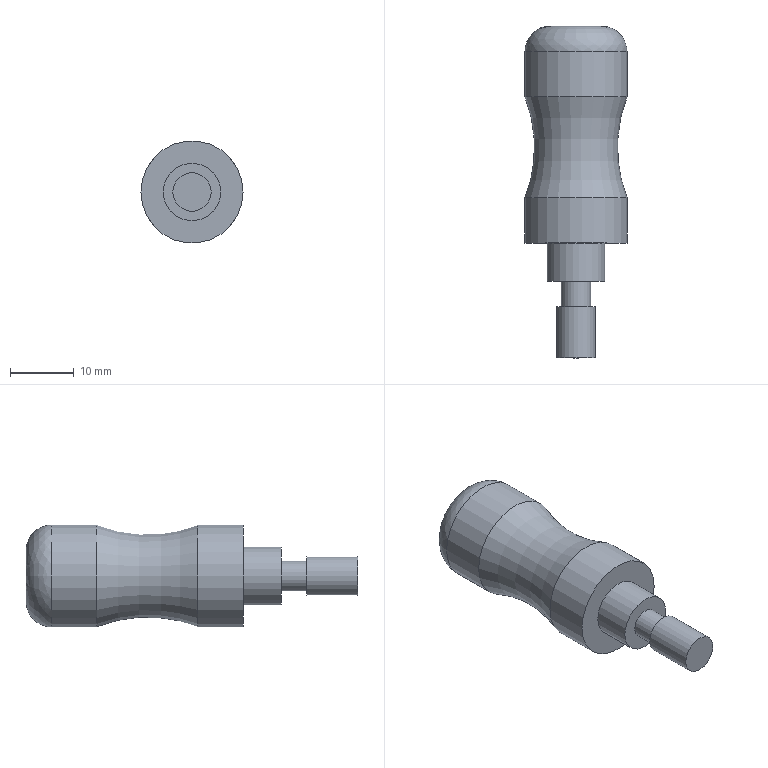Component | NX | 11_HANDLE | 1 solid | 12 faces | box 16 x 52 x 16 mm | volume 6616 mm3 | cylinder 5 | plane 5 | torus 1 | spline 1 | commonest cylinder face diameters 16 x2 9 x1 4.6 x1 6 x1
STEP:
#1=CARTESIAN_POINT('',(0.,0.,0.));
#2=DIRECTION('',(0.,0.,1.));
#3=DIRECTION('',(1.,0.,0.));
#4=AXIS2_PLACEMENT_3D('',#1,#2,#3);
#5=CARTESIAN_POINT('',(10.02,86.13,15.172));
#6=VERTEX_POINT('',#5);
#7=CARTESIAN_POINT('',(2.02,86.13,15.172));
#8=DIRECTION('',(0.,1.,0.));
#9=DIRECTION('',(1.,0.,0.));
#10=AXIS2_PLACEMENT_3D('',#7,#8,#9);
#11=CIRCLE('',#10,8.);
#12=CARTESIAN_POINT('',(2.02,120.13,15.172));
#13=DIRECTION('',(0.,-1.,0.));
#14=DIRECTION('',(1.,0.,0.));
#15=AXIS2_PLACEMENT_3D('',#12,#13,#14);
#16=CYLINDRICAL_SURFACE('',#15,8.);
#17=CARTESIAN_POINT('',(6.283,34.));
#18=DIRECTION('',(-1.,0.));
#19=VECTOR('',#18,1.);
#20=LINE('',#17,#19);
#21=(GEOMETRIC_REPRESENTATION_CONTEXT(2)PARAMETRIC_REPRESENTATION_CONTEXT()REPRESENTATION_CONTEXT('',''));
#22=DEFINITIONAL_REPRESENTATION('',(#20),#21);
#23=PCURVE('',#16,#22);
#24=CARTESIAN_POINT('',(2.02,86.13,15.172));
#25=DIRECTION('',(0.,-1.,0.));
#26=DIRECTION('',(1.,0.,0.));
#27=AXIS2_PLACEMENT_3D('',#24,#25,#26);
#28=PLANE('',#27);
#29=CARTESIAN_POINT('',(8.,0.));
#30=CARTESIAN_POINT('',(8.,-13.856));
#31=CARTESIAN_POINT('',(-4.,-6.928));
#32=CARTESIAN_POINT('',(-16.,-0.));
#33=CARTESIAN_POINT('',(-4.,6.928));
#34=CARTESIAN_POINT('',(8.,13.856));
#35=CARTESIAN_POINT('',(8.,0.));
#36=(BOUNDED_CURVE()B_SPLINE_CURVE(2,(#29,#30,#31,#32,#33,#34,#35),.UNSPECIFIED.,.T.,.F.)B_SPLINE_CURVE_WITH_KNOTS((1,2,2,2,2,1),(-2.094,0.,2.094,4.189,6.283,8.378),.UNSPECIFIED.)CURVE()GEOMETRIC_REPRESENTATION_ITEM()RATIONAL_B_SPLINE_CURVE((1.,0.5,1.,0.5,1.,0.5,1.))REPRESENTATION_ITEM(''));
#37=(GEOMETRIC_REPRESENTATION_CONTEXT(2)PARAMETRIC_REPRESENTATION_CONTEXT()REPRESENTATION_CONTEXT('',''));
#38=DEFINITIONAL_REPRESENTATION('',(#36),#37);
#39=PCURVE('',#28,#38);
#40=SURFACE_CURVE('',#11,(#23,#39),.PCURVE_S1.);
#41=EDGE_CURVE('',#6,#6,#40,.T.);
#42=ORIENTED_EDGE('',*,*,#41,.T.);
#43=CARTESIAN_POINT('',(10.02,93.23,15.172));
#44=VERTEX_POINT('',#43);
#45=CARTESIAN_POINT('',(10.02,93.23,15.172));
#46=CARTESIAN_POINT('',(10.02,86.13,15.172));
#47=B_SPLINE_CURVE_WITH_KNOTS('',1,(#45,#46),.UNSPECIFIED.,.F.,.F.,(2,2),(26.9,34.),.PIECEWISE_BEZIER_KNOTS.);
#48=CARTESIAN_POINT('',(0.,0.));
#49=DIRECTION('',(0.,1.));
#50=VECTOR('',#49,1.);
#51=LINE('',#48,#50);
#52=(GEOMETRIC_REPRESENTATION_CONTEXT(2)PARAMETRIC_REPRESENTATION_CONTEXT()REPRESENTATION_CONTEXT('',''));
#53=DEFINITIONAL_REPRESENTATION('',(#51),#52);
#54=PCURVE('',#16,#53);
#55=CARTESIAN_POINT('',(6.283,0.));
#56=DIRECTION('',(0.,1.));
#57=VECTOR('',#56,1.);
#58=LINE('',#55,#57);
#59=(GEOMETRIC_REPRESENTATION_CONTEXT(2)PARAMETRIC_REPRESENTATION_CONTEXT()REPRESENTATION_CONTEXT('',''));
#60=DEFINITIONAL_REPRESENTATION('',(#58),#59);
#61=PCURVE('',#16,#60);
#62=SEAM_CURVE('',#47,(#54,#61),.PCURVE_S1.);
#63=EDGE_CURVE('',#44,#6,#62,.T.);
#64=ORIENTED_EDGE('',*,*,#63,.F.);
#65=CARTESIAN_POINT('',(-5.98,93.23,15.172));
#66=VERTEX_POINT('',#65);
#67=CARTESIAN_POINT('',(2.02,93.23,15.172));
#68=DIRECTION('',(0.,-1.,0.));
#69=DIRECTION('',(-1.,0.,0.));
#70=AXIS2_PLACEMENT_3D('',#67,#68,#69);
#71=CIRCLE('',#70,8.);
#72=CARTESIAN_POINT('',(-3.142,26.9));
#73=DIRECTION('',(1.,0.));
#74=VECTOR('',#73,1.);
#75=LINE('',#72,#74);
#76=(GEOMETRIC_REPRESENTATION_CONTEXT(2)PARAMETRIC_REPRESENTATION_CONTEXT()REPRESENTATION_CONTEXT('',''));
#77=DEFINITIONAL_REPRESENTATION('',(#75),#76);
#78=PCURVE('',#16,#77);
#79=CARTESIAN_POINT('',(2.02,101.13,15.172));
#80=DIRECTION('',(0.,1.,0.));
#81=DIRECTION('',(-1.,0.,0.));
#82=AXIS2_PLACEMENT_3D('',#79,#80,#81);
#83=TOROIDAL_SURFACE('',#82,28.053,21.553);
#84=CARTESIAN_POINT('',(6.283,3.517));
#85=DIRECTION('',(-1.,0.));
#86=VECTOR('',#85,1.);
#87=LINE('',#84,#86);
#88=(GEOMETRIC_REPRESENTATION_CONTEXT(2)PARAMETRIC_REPRESENTATION_CONTEXT()REPRESENTATION_CONTEXT('',''));
#89=DEFINITIONAL_REPRESENTATION('',(#87),#88);
#90=PCURVE('',#83,#89);
#91=SURFACE_CURVE('',#71,(#78,#90),.PCURVE_S1.);
#92=EDGE_CURVE('',#44,#66,#91,.T.);
#93=ORIENTED_EDGE('',*,*,#92,.T.);
#94=CARTESIAN_POINT('',(2.02,93.23,15.172));
#95=DIRECTION('',(0.,-1.,0.));
#96=DIRECTION('',(-1.,0.,0.));
#97=AXIS2_PLACEMENT_3D('',#94,#95,#96);
#98=CIRCLE('',#97,8.);
#99=CARTESIAN_POINT('',(3.142,26.9));
#100=DIRECTION('',(1.,0.));
#101=VECTOR('',#100,1.);
#102=LINE('',#99,#101);
#103=(GEOMETRIC_REPRESENTATION_CONTEXT(2)PARAMETRIC_REPRESENTATION_CONTEXT()REPRESENTATION_CONTEXT('',''));
#104=DEFINITIONAL_REPRESENTATION('',(#102),#103);
#105=PCURVE('',#16,#104);
#106=CARTESIAN_POINT('',(6.283,3.517));
#107=DIRECTION('',(-1.,0.));
#108=VECTOR('',#107,1.);
#109=LINE('',#106,#108);
#110=(GEOMETRIC_REPRESENTATION_CONTEXT(2)PARAMETRIC_REPRESENTATION_CONTEXT()REPRESENTATION_CONTEXT('',''));
#111=DEFINITIONAL_REPRESENTATION('',(#109),#110);
#112=PCURVE('',#83,#111);
#113=SURFACE_CURVE('',#98,(#105,#112),.PCURVE_S1.);
#114=EDGE_CURVE('',#66,#44,#113,.T.);
#115=ORIENTED_EDGE('',*,*,#114,.T.);
#116=ORIENTED_EDGE('',*,*,#63,.T.);
#117=EDGE_LOOP('',(#42,#64,#93,#115,#116));
#118=FACE_BOUND('',#117,.T.);
#119=ADVANCED_FACE('',(#118),#16,.T.);
#120=CARTESIAN_POINT('',(6.52,86.13,15.172));
#121=VERTEX_POINT('',#120);
#122=CARTESIAN_POINT('',(2.02,86.13,15.172));
#123=DIRECTION('',(0.,-1.,0.));
#124=DIRECTION('',(1.,0.,0.));
#125=AXIS2_PLACEMENT_3D('',#122,#123,#124);
#126=CIRCLE('',#125,4.5);
#127=CARTESIAN_POINT('',(0.,0.));
#128=DIRECTION('',(1.,0.));
#129=AXIS2_PLACEMENT_2D('',#127,#128);
#130=CIRCLE('',#129,4.5);
#131=(GEOMETRIC_REPRESENTATION_CONTEXT(2)PARAMETRIC_REPRESENTATION_CONTEXT()REPRESENTATION_CONTEXT('',''));
#132=DEFINITIONAL_REPRESENTATION('',(#130),#131);
#133=PCURVE('',#28,#132);
#134=CARTESIAN_POINT('',(2.02,86.13,15.172));
#135=DIRECTION('',(0.,-1.,0.));
#136=DIRECTION('',(1.,0.,0.));
#137=AXIS2_PLACEMENT_3D('',#134,#135,#136);
#138=CYLINDRICAL_SURFACE('',#137,4.5);
#139=CARTESIAN_POINT('',(0.,0.));
#140=DIRECTION('',(1.,0.));
#141=VECTOR('',#140,1.);
#142=LINE('',#139,#141);
#143=(GEOMETRIC_REPRESENTATION_CONTEXT(2)PARAMETRIC_REPRESENTATION_CONTEXT()REPRESENTATION_CONTEXT('',''));
#144=DEFINITIONAL_REPRESENTATION('',(#142),#143);
#145=PCURVE('',#138,#144);
#146=SURFACE_CURVE('',#126,(#133,#145),.PCURVE_S1.);
#147=EDGE_CURVE('',#121,#121,#146,.T.);
#148=ORIENTED_EDGE('',*,*,#147,.F.);
#149=EDGE_LOOP('',(#148));
#150=FACE_BOUND('',#149,.T.);
#151=ORIENTED_EDGE('',*,*,#41,.F.);
#152=EDGE_LOOP('',(#151));
#153=FACE_BOUND('',#152,.T.);
#154=ADVANCED_FACE('',(#150,#153),#28,.T.);
#155=CARTESIAN_POINT('',(4.32,80.13,15.172));
#156=VERTEX_POINT('',#155);
#157=CARTESIAN_POINT('',(2.02,80.13,15.172));
#158=DIRECTION('',(0.,-1.,0.));
#159=DIRECTION('',(1.,0.,0.));
#160=AXIS2_PLACEMENT_3D('',#157,#158,#159);
#161=CIRCLE('',#160,2.3);
#162=CARTESIAN_POINT('',(2.02,80.13,15.172));
#163=DIRECTION('',(0.,-1.,0.));
#164=DIRECTION('',(1.,0.,0.));
#165=AXIS2_PLACEMENT_3D('',#162,#163,#164);
#166=PLANE('',#165);
#167=CARTESIAN_POINT('',(0.,0.));
#168=DIRECTION('',(1.,0.));
#169=AXIS2_PLACEMENT_2D('',#167,#168);
#170=CIRCLE('',#169,2.3);
#171=(GEOMETRIC_REPRESENTATION_CONTEXT(2)PARAMETRIC_REPRESENTATION_CONTEXT()REPRESENTATION_CONTEXT('',''));
#172=DEFINITIONAL_REPRESENTATION('',(#170),#171);
#173=PCURVE('',#166,#172);
#174=CARTESIAN_POINT('',(2.02,80.13,15.172));
#175=DIRECTION('',(0.,-1.,0.));
#176=DIRECTION('',(1.,0.,0.));
#177=AXIS2_PLACEMENT_3D('',#174,#175,#176);
#178=CYLINDRICAL_SURFACE('',#177,2.3);
#179=CARTESIAN_POINT('',(0.,0.));
#180=DIRECTION('',(1.,0.));
#181=VECTOR('',#180,1.);
#182=LINE('',#179,#181);
#183=(GEOMETRIC_REPRESENTATION_CONTEXT(2)PARAMETRIC_REPRESENTATION_CONTEXT()REPRESENTATION_CONTEXT('',''));
#184=DEFINITIONAL_REPRESENTATION('',(#182),#183);
#185=PCURVE('',#178,#184);
#186=SURFACE_CURVE('',#161,(#173,#185),.PCURVE_S1.);
#187=EDGE_CURVE('',#156,#156,#186,.T.);
#188=ORIENTED_EDGE('',*,*,#187,.F.);
#189=EDGE_LOOP('',(#188));
#190=FACE_BOUND('',#189,.T.);
#191=CARTESIAN_POINT('',(6.52,80.13,15.172));
#192=VERTEX_POINT('',#191);
#193=CARTESIAN_POINT('',(2.02,80.13,15.172));
#194=DIRECTION('',(0.,1.,0.));
#195=DIRECTION('',(1.,0.,0.));
#196=AXIS2_PLACEMENT_3D('',#193,#194,#195);
#197=CIRCLE('',#196,4.5);
#198=CARTESIAN_POINT('',(4.5,0.));
#199=CARTESIAN_POINT('',(4.5,-7.794));
#200=CARTESIAN_POINT('',(-2.25,-3.897));
#201=CARTESIAN_POINT('',(-9.,-0.));
#202=CARTESIAN_POINT('',(-2.25,3.897));
#203=CARTESIAN_POINT('',(4.5,7.794));
#204=CARTESIAN_POINT('',(4.5,0.));
#205=(BOUNDED_CURVE()B_SPLINE_CURVE(2,(#198,#199,#200,#201,#202,#203,#204),.UNSPECIFIED.,.T.,.F.)B_SPLINE_CURVE_WITH_KNOTS((1,2,2,2,2,1),(-2.094,0.,2.094,4.189,6.283,8.378),.UNSPECIFIED.)CURVE()GEOMETRIC_REPRESENTATION_ITEM()RATIONAL_B_SPLINE_CURVE((1.,0.5,1.,0.5,1.,0.5,1.))REPRESENTATION_ITEM(''));
#206=(GEOMETRIC_REPRESENTATION_CONTEXT(2)PARAMETRIC_REPRESENTATION_CONTEXT()REPRESENTATION_CONTEXT('',''));
#207=DEFINITIONAL_REPRESENTATION('',(#205),#206);
#208=PCURVE('',#166,#207);
#209=CARTESIAN_POINT('',(6.283,6.));
#210=DIRECTION('',(-1.,0.));
#211=VECTOR('',#210,1.);
#212=LINE('',#209,#211);
#213=(GEOMETRIC_REPRESENTATION_CONTEXT(2)PARAMETRIC_REPRESENTATION_CONTEXT()REPRESENTATION_CONTEXT('',''));
#214=DEFINITIONAL_REPRESENTATION('',(#212),#213);
#215=PCURVE('',#138,#214);
#216=SURFACE_CURVE('',#197,(#208,#215),.PCURVE_S1.);
#217=EDGE_CURVE('',#192,#192,#216,.T.);
#218=ORIENTED_EDGE('',*,*,#217,.F.);
#219=EDGE_LOOP('',(#218));
#220=FACE_BOUND('',#219,.T.);
#221=ADVANCED_FACE('',(#190,#220),#166,.T.);
#222=ORIENTED_EDGE('',*,*,#217,.T.);
#223=CARTESIAN_POINT('',(6.52,86.13,15.172));
#224=CARTESIAN_POINT('',(6.52,80.13,15.172));
#225=B_SPLINE_CURVE_WITH_KNOTS('',1,(#223,#224),.UNSPECIFIED.,.F.,.F.,(2,2),(0.,6.),.PIECEWISE_BEZIER_KNOTS.);
#226=CARTESIAN_POINT('',(0.,0.));
#227=DIRECTION('',(0.,1.));
#228=VECTOR('',#227,1.);
#229=LINE('',#226,#228);
#230=(GEOMETRIC_REPRESENTATION_CONTEXT(2)PARAMETRIC_REPRESENTATION_CONTEXT()REPRESENTATION_CONTEXT('',''));
#231=DEFINITIONAL_REPRESENTATION('',(#229),#230);
#232=PCURVE('',#138,#231);
#233=CARTESIAN_POINT('',(6.283,0.));
#234=DIRECTION('',(0.,1.));
#235=VECTOR('',#234,1.);
#236=LINE('',#233,#235);
#237=(GEOMETRIC_REPRESENTATION_CONTEXT(2)PARAMETRIC_REPRESENTATION_CONTEXT()REPRESENTATION_CONTEXT('',''));
#238=DEFINITIONAL_REPRESENTATION('',(#236),#237);
#239=PCURVE('',#138,#238);
#240=SEAM_CURVE('',#225,(#232,#239),.PCURVE_S1.);
#241=EDGE_CURVE('',#121,#192,#240,.T.);
#242=ORIENTED_EDGE('',*,*,#241,.F.);
#243=ORIENTED_EDGE('',*,*,#147,.T.);
#244=ORIENTED_EDGE('',*,*,#241,.T.);
#245=EDGE_LOOP('',(#222,#242,#243,#244));
#246=FACE_BOUND('',#245,.T.);
#247=ADVANCED_FACE('',(#246),#138,.T.);
#248=CARTESIAN_POINT('',(4.32,76.13,15.172));
#249=VERTEX_POINT('',#248);
#250=CARTESIAN_POINT('',(-0.2796,76.13,15.172));
#251=VERTEX_POINT('',#250);
#252=CARTESIAN_POINT('',(2.02,76.13,15.172));
#253=DIRECTION('',(0.,-1.,0.));
#254=DIRECTION('',(-1.,0.,0.));
#255=AXIS2_PLACEMENT_3D('',#252,#253,#254);
#256=CIRCLE('',#255,2.3);
#257=CARTESIAN_POINT('',(-3.142,4.));
#258=DIRECTION('',(1.,0.));
#259=VECTOR('',#258,1.);
#260=LINE('',#257,#259);
#261=(GEOMETRIC_REPRESENTATION_CONTEXT(2)PARAMETRIC_REPRESENTATION_CONTEXT()REPRESENTATION_CONTEXT('',''));
#262=DEFINITIONAL_REPRESENTATION('',(#260),#261);
#263=PCURVE('',#178,#262);
#264=CARTESIAN_POINT('',(2.02,76.13,15.172));
#265=DIRECTION('',(0.,1.,0.));
#266=DIRECTION('',(-1.,0.,0.));
#267=AXIS2_PLACEMENT_3D('',#264,#265,#266);
#268=PLANE('',#267);
#269=CARTESIAN_POINT('',(2.3,0.));
#270=CARTESIAN_POINT('',(2.3,-3.984));
#271=CARTESIAN_POINT('',(-1.15,-1.992));
#272=CARTESIAN_POINT('',(-4.6,-0.));
#273=CARTESIAN_POINT('',(-1.15,1.992));
#274=CARTESIAN_POINT('',(2.3,3.984));
#275=CARTESIAN_POINT('',(2.3,0.));
#276=(BOUNDED_CURVE()B_SPLINE_CURVE(2,(#269,#270,#271,#272,#273,#274,#275),.UNSPECIFIED.,.T.,.F.)B_SPLINE_CURVE_WITH_KNOTS((1,2,2,2,2,1),(-2.094,0.,2.094,4.189,6.283,8.378),.UNSPECIFIED.)CURVE()GEOMETRIC_REPRESENTATION_ITEM()RATIONAL_B_SPLINE_CURVE((1.,0.5,1.,0.5,1.,0.5,1.))REPRESENTATION_ITEM(''));
#277=(GEOMETRIC_REPRESENTATION_CONTEXT(2)PARAMETRIC_REPRESENTATION_CONTEXT()REPRESENTATION_CONTEXT('',''));
#278=DEFINITIONAL_REPRESENTATION('',(#276),#277);
#279=PCURVE('',#268,#278);
#280=SURFACE_CURVE('',#256,(#263,#279),.PCURVE_S1.);
#281=EDGE_CURVE('',#249,#251,#280,.T.);
#282=ORIENTED_EDGE('',*,*,#281,.F.);
#283=CARTESIAN_POINT('',(4.32,80.13,15.172));
#284=CARTESIAN_POINT('',(4.32,76.13,15.172));
#285=B_SPLINE_CURVE_WITH_KNOTS('',1,(#283,#284),.UNSPECIFIED.,.F.,.F.,(2,2),(0.,4.),.PIECEWISE_BEZIER_KNOTS.);
#286=CARTESIAN_POINT('',(0.,0.));
#287=DIRECTION('',(0.,1.));
#288=VECTOR('',#287,1.);
#289=LINE('',#286,#288);
#290=(GEOMETRIC_REPRESENTATION_CONTEXT(2)PARAMETRIC_REPRESENTATION_CONTEXT()REPRESENTATION_CONTEXT('',''));
#291=DEFINITIONAL_REPRESENTATION('',(#289),#290);
#292=PCURVE('',#178,#291);
#293=CARTESIAN_POINT('',(6.283,0.));
#294=DIRECTION('',(0.,1.));
#295=VECTOR('',#294,1.);
#296=LINE('',#293,#295);
#297=(GEOMETRIC_REPRESENTATION_CONTEXT(2)PARAMETRIC_REPRESENTATION_CONTEXT()REPRESENTATION_CONTEXT('',''));
#298=DEFINITIONAL_REPRESENTATION('',(#296),#297);
#299=PCURVE('',#178,#298);
#300=SEAM_CURVE('',#285,(#292,#299),.PCURVE_S1.);
#301=EDGE_CURVE('',#156,#249,#300,.T.);
#302=ORIENTED_EDGE('',*,*,#301,.F.);
#303=ORIENTED_EDGE('',*,*,#187,.T.);
#304=ORIENTED_EDGE('',*,*,#301,.T.);
#305=CARTESIAN_POINT('',(2.02,76.13,15.172));
#306=DIRECTION('',(0.,-1.,0.));
#307=DIRECTION('',(-1.,0.,0.));
#308=AXIS2_PLACEMENT_3D('',#305,#306,#307);
#309=CIRCLE('',#308,2.3);
#310=CARTESIAN_POINT('',(3.142,4.));
#311=DIRECTION('',(1.,0.));
#312=VECTOR('',#311,1.);
#313=LINE('',#310,#312);
#314=(GEOMETRIC_REPRESENTATION_CONTEXT(2)PARAMETRIC_REPRESENTATION_CONTEXT()REPRESENTATION_CONTEXT('',''));
#315=DEFINITIONAL_REPRESENTATION('',(#313),#314);
#316=PCURVE('',#178,#315);
#317=CARTESIAN_POINT('',(2.3,0.));
#318=CARTESIAN_POINT('',(2.3,-3.984));
#319=CARTESIAN_POINT('',(-1.15,-1.992));
#320=CARTESIAN_POINT('',(-4.6,-0.));
#321=CARTESIAN_POINT('',(-1.15,1.992));
#322=CARTESIAN_POINT('',(2.3,3.984));
#323=CARTESIAN_POINT('',(2.3,0.));
#324=(BOUNDED_CURVE()B_SPLINE_CURVE(2,(#317,#318,#319,#320,#321,#322,#323),.UNSPECIFIED.,.T.,.F.)B_SPLINE_CURVE_WITH_KNOTS((1,2,2,2,2,1),(-2.094,0.,2.094,4.189,6.283,8.378),.UNSPECIFIED.)CURVE()GEOMETRIC_REPRESENTATION_ITEM()RATIONAL_B_SPLINE_CURVE((1.,0.5,1.,0.5,1.,0.5,1.))REPRESENTATION_ITEM(''));
#325=(GEOMETRIC_REPRESENTATION_CONTEXT(2)PARAMETRIC_REPRESENTATION_CONTEXT()REPRESENTATION_CONTEXT('',''));
#326=DEFINITIONAL_REPRESENTATION('',(#324),#325);
#327=PCURVE('',#268,#326);
#328=SURFACE_CURVE('',#309,(#316,#327),.PCURVE_S1.);
#329=EDGE_CURVE('',#251,#249,#328,.T.);
#330=ORIENTED_EDGE('',*,*,#329,.F.);
#331=EDGE_LOOP('',(#282,#302,#303,#304,#330));
#332=FACE_BOUND('',#331,.T.);
#333=ADVANCED_FACE('',(#332),#178,.T.);
#334=CARTESIAN_POINT('',(5.02,68.13,15.172));
#335=VERTEX_POINT('',#334);
#336=CARTESIAN_POINT('',(2.02,68.13,15.172));
#337=DIRECTION('',(0.,1.,0.));
#338=DIRECTION('',(1.,0.,0.));
#339=AXIS2_PLACEMENT_3D('',#336,#337,#338);
#340=CIRCLE('',#339,3.);
#341=CARTESIAN_POINT('',(2.02,68.13,15.172));
#342=DIRECTION('',(0.,-1.,0.));
#343=DIRECTION('',(1.,0.,0.));
#344=AXIS2_PLACEMENT_3D('',#341,#342,#343);
#345=PLANE('',#344);
#346=CARTESIAN_POINT('',(3.,0.));
#347=CARTESIAN_POINT('',(3.,-5.196));
#348=CARTESIAN_POINT('',(-1.5,-2.598));
#349=CARTESIAN_POINT('',(-6.,-0.));
#350=CARTESIAN_POINT('',(-1.5,2.598));
#351=CARTESIAN_POINT('',(3.,5.196));
#352=CARTESIAN_POINT('',(3.,0.));
#353=(BOUNDED_CURVE()B_SPLINE_CURVE(2,(#346,#347,#348,#349,#350,#351,#352),.UNSPECIFIED.,.T.,.F.)B_SPLINE_CURVE_WITH_KNOTS((1,2,2,2,2,1),(-2.094,0.,2.094,4.189,6.283,8.378),.UNSPECIFIED.)CURVE()GEOMETRIC_REPRESENTATION_ITEM()RATIONAL_B_SPLINE_CURVE((1.,0.5,1.,0.5,1.,0.5,1.))REPRESENTATION_ITEM(''));
#354=(GEOMETRIC_REPRESENTATION_CONTEXT(2)PARAMETRIC_REPRESENTATION_CONTEXT()REPRESENTATION_CONTEXT('',''));
#355=DEFINITIONAL_REPRESENTATION('',(#353),#354);
#356=PCURVE('',#345,#355);
#357=CARTESIAN_POINT('',(2.02,76.13,15.172));
#358=DIRECTION('',(0.,-1.,0.));
#359=DIRECTION('',(1.,0.,0.));
#360=AXIS2_PLACEMENT_3D('',#357,#358,#359);
#361=CYLINDRICAL_SURFACE('',#360,3.);
#362=CARTESIAN_POINT('',(6.283,8.));
#363=DIRECTION('',(-1.,0.));
#364=VECTOR('',#363,1.);
#365=LINE('',#362,#364);
#366=(GEOMETRIC_REPRESENTATION_CONTEXT(2)PARAMETRIC_REPRESENTATION_CONTEXT()REPRESENTATION_CONTEXT('',''));
#367=DEFINITIONAL_REPRESENTATION('',(#365),#366);
#368=PCURVE('',#361,#367);
#369=SURFACE_CURVE('',#340,(#356,#368),.PCURVE_S1.);
#370=EDGE_CURVE('',#335,#335,#369,.T.);
#371=ORIENTED_EDGE('',*,*,#370,.F.);
#372=EDGE_LOOP('',(#371));
#373=FACE_BOUND('',#372,.T.);
#374=ADVANCED_FACE('',(#373),#345,.T.);
#375=ORIENTED_EDGE('',*,*,#329,.T.);
#376=ORIENTED_EDGE('',*,*,#281,.T.);
#377=EDGE_LOOP('',(#375,#376));
#378=FACE_BOUND('',#377,.T.);
#379=CARTESIAN_POINT('',(5.02,76.13,15.172));
#380=VERTEX_POINT('',#379);
#381=CARTESIAN_POINT('',(2.02,76.13,15.172));
#382=DIRECTION('',(0.,-1.,0.));
#383=DIRECTION('',(1.,0.,0.));
#384=AXIS2_PLACEMENT_3D('',#381,#382,#383);
#385=CIRCLE('',#384,3.);
#386=CARTESIAN_POINT('',(-3.,0.));
#387=CARTESIAN_POINT('',(-3.,5.196));
#388=CARTESIAN_POINT('',(1.5,2.598));
#389=CARTESIAN_POINT('',(6.,0.));
#390=CARTESIAN_POINT('',(1.5,-2.598));
#391=CARTESIAN_POINT('',(-3.,-5.196));
#392=CARTESIAN_POINT('',(-3.,0.));
#393=(BOUNDED_CURVE()B_SPLINE_CURVE(2,(#386,#387,#388,#389,#390,#391,#392),.UNSPECIFIED.,.T.,.F.)B_SPLINE_CURVE_WITH_KNOTS((1,2,2,2,2,1),(-2.094,0.,2.094,4.189,6.283,8.378),.UNSPECIFIED.)CURVE()GEOMETRIC_REPRESENTATION_ITEM()RATIONAL_B_SPLINE_CURVE((1.,0.5,1.,0.5,1.,0.5,1.))REPRESENTATION_ITEM(''));
#394=(GEOMETRIC_REPRESENTATION_CONTEXT(2)PARAMETRIC_REPRESENTATION_CONTEXT()REPRESENTATION_CONTEXT('',''));
#395=DEFINITIONAL_REPRESENTATION('',(#393),#394);
#396=PCURVE('',#268,#395);
#397=CARTESIAN_POINT('',(0.,0.));
#398=DIRECTION('',(1.,0.));
#399=VECTOR('',#398,1.);
#400=LINE('',#397,#399);
#401=(GEOMETRIC_REPRESENTATION_CONTEXT(2)PARAMETRIC_REPRESENTATION_CONTEXT()REPRESENTATION_CONTEXT('',''));
#402=DEFINITIONAL_REPRESENTATION('',(#400),#401);
#403=PCURVE('',#361,#402);
#404=SURFACE_CURVE('',#385,(#396,#403),.PCURVE_S1.);
#405=EDGE_CURVE('',#380,#380,#404,.T.);
#406=ORIENTED_EDGE('',*,*,#405,.F.);
#407=EDGE_LOOP('',(#406));
#408=FACE_BOUND('',#407,.T.);
#409=ADVANCED_FACE('',(#378,#408),#268,.T.);
#410=ORIENTED_EDGE('',*,*,#370,.T.);
#411=CARTESIAN_POINT('',(5.02,76.13,15.172));
#412=CARTESIAN_POINT('',(5.02,68.13,15.172));
#413=B_SPLINE_CURVE_WITH_KNOTS('',1,(#411,#412),.UNSPECIFIED.,.F.,.F.,(2,2),(0.,8.),.PIECEWISE_BEZIER_KNOTS.);
#414=CARTESIAN_POINT('',(0.,0.));
#415=DIRECTION('',(0.,1.));
#416=VECTOR('',#415,1.);
#417=LINE('',#414,#416);
#418=(GEOMETRIC_REPRESENTATION_CONTEXT(2)PARAMETRIC_REPRESENTATION_CONTEXT()REPRESENTATION_CONTEXT('',''));
#419=DEFINITIONAL_REPRESENTATION('',(#417),#418);
#420=PCURVE('',#361,#419);
#421=CARTESIAN_POINT('',(6.283,0.));
#422=DIRECTION('',(0.,1.));
#423=VECTOR('',#422,1.);
#424=LINE('',#421,#423);
#425=(GEOMETRIC_REPRESENTATION_CONTEXT(2)PARAMETRIC_REPRESENTATION_CONTEXT()REPRESENTATION_CONTEXT('',''));
#426=DEFINITIONAL_REPRESENTATION('',(#424),#425);
#427=PCURVE('',#361,#426);
#428=SEAM_CURVE('',#413,(#420,#427),.PCURVE_S1.);
#429=EDGE_CURVE('',#380,#335,#428,.T.);
#430=ORIENTED_EDGE('',*,*,#429,.F.);
#431=ORIENTED_EDGE('',*,*,#405,.T.);
#432=ORIENTED_EDGE('',*,*,#429,.T.);
#433=EDGE_LOOP('',(#410,#430,#431,#432));
#434=FACE_BOUND('',#433,.T.);
#435=ADVANCED_FACE('',(#434),#361,.T.);
#436=ORIENTED_EDGE('',*,*,#92,.T.);
#437=CARTESIAN_POINT('',(-5.98,109.03,15.172));
#438=VERTEX_POINT('',#437);
#439=CARTESIAN_POINT('',(-5.98,109.03,15.172));
#440=CARTESIAN_POINT('',(-4.987,106.51,15.172));
#441=CARTESIAN_POINT('',(-4.379,103.855,15.172));
#442=CARTESIAN_POINT('',(-4.174,101.13,15.172));
#443=CARTESIAN_POINT('',(-4.379,98.406,15.172));
#444=CARTESIAN_POINT('',(-4.987,95.751,15.172));
#445=CARTESIAN_POINT('',(-5.98,93.23,15.172));
#446=(BOUNDED_CURVE()B_SPLINE_CURVE(6,(#439,#440,#441,#442,#443,#444,#445),.UNSPECIFIED.,.F.,.F.)B_SPLINE_CURVE_WITH_KNOTS((7,7),(2.766,3.517),.PIECEWISE_BEZIER_KNOTS.)CURVE()GEOMETRIC_REPRESENTATION_ITEM()RATIONAL_B_SPLINE_CURVE((1.007,1.002,0.9995,0.9986,0.9995,1.002,1.007))REPRESENTATION_ITEM(''));
#447=CARTESIAN_POINT('',(0.,0.));
#448=DIRECTION('',(0.,1.));
#449=VECTOR('',#448,1.);
#450=LINE('',#447,#449);
#451=(GEOMETRIC_REPRESENTATION_CONTEXT(2)PARAMETRIC_REPRESENTATION_CONTEXT()REPRESENTATION_CONTEXT('',''));
#452=DEFINITIONAL_REPRESENTATION('',(#450),#451);
#453=PCURVE('',#83,#452);
#454=CARTESIAN_POINT('',(6.283,0.));
#455=DIRECTION('',(0.,1.));
#456=VECTOR('',#455,1.);
#457=LINE('',#454,#456);
#458=(GEOMETRIC_REPRESENTATION_CONTEXT(2)PARAMETRIC_REPRESENTATION_CONTEXT()REPRESENTATION_CONTEXT('',''));
#459=DEFINITIONAL_REPRESENTATION('',(#457),#458);
#460=PCURVE('',#83,#459);
#461=SEAM_CURVE('',#446,(#453,#460),.PCURVE_S1.);
#462=EDGE_CURVE('',#438,#66,#461,.T.);
#463=ORIENTED_EDGE('',*,*,#462,.F.);
#464=CARTESIAN_POINT('',(2.02,109.03,15.172));
#465=DIRECTION('',(0.,1.,0.));
#466=DIRECTION('',(-1.,0.,0.));
#467=AXIS2_PLACEMENT_3D('',#464,#465,#466);
#468=CIRCLE('',#467,8.);
#469=CARTESIAN_POINT('',(0.,2.766));
#470=DIRECTION('',(1.,0.));
#471=VECTOR('',#470,1.);
#472=LINE('',#469,#471);
#473=(GEOMETRIC_REPRESENTATION_CONTEXT(2)PARAMETRIC_REPRESENTATION_CONTEXT()REPRESENTATION_CONTEXT('',''));
#474=DEFINITIONAL_REPRESENTATION('',(#472),#473);
#475=PCURVE('',#83,#474);
#476=CARTESIAN_POINT('',(2.02,120.13,15.172));
#477=DIRECTION('',(0.,-1.,0.));
#478=DIRECTION('',(1.,0.,0.));
#479=AXIS2_PLACEMENT_3D('',#476,#477,#478);
#480=CYLINDRICAL_SURFACE('',#479,8.);
#481=CARTESIAN_POINT('',(9.425,11.1));
#482=DIRECTION('',(-1.,0.));
#483=VECTOR('',#482,1.);
#484=LINE('',#481,#483);
#485=(GEOMETRIC_REPRESENTATION_CONTEXT(2)PARAMETRIC_REPRESENTATION_CONTEXT()REPRESENTATION_CONTEXT('',''));
#486=DEFINITIONAL_REPRESENTATION('',(#484),#485);
#487=PCURVE('',#480,#486);
#488=SURFACE_CURVE('',#468,(#475,#487),.PCURVE_S1.);
#489=EDGE_CURVE('',#438,#438,#488,.T.);
#490=ORIENTED_EDGE('',*,*,#489,.T.);
#491=ORIENTED_EDGE('',*,*,#462,.T.);
#492=ORIENTED_EDGE('',*,*,#114,.T.);
#493=EDGE_LOOP('',(#436,#463,#490,#491,#492));
#494=FACE_BOUND('',#493,.F.);
#495=ADVANCED_FACE('',(#494),#83,.F.);
#496=CARTESIAN_POINT('',(-1.98,120.13,15.172));
#497=VERTEX_POINT('',#496);
#498=CARTESIAN_POINT('',(2.02,120.13,15.172));
#499=DIRECTION('',(0.,1.,0.));
#500=DIRECTION('',(-1.,0.,0.));
#501=AXIS2_PLACEMENT_3D('',#498,#499,#500);
#502=CIRCLE('',#501,4.);
#503=CARTESIAN_POINT('',(2.02,120.13,15.172));
#504=DIRECTION('',(0.,1.,0.));
#505=DIRECTION('',(-1.,0.,0.));
#506=AXIS2_PLACEMENT_3D('',#503,#504,#505);
#507=PLANE('',#506);
#508=CARTESIAN_POINT('',(0.,0.));
#509=DIRECTION('',(1.,0.));
#510=AXIS2_PLACEMENT_2D('',#508,#509);
#511=CIRCLE('',#510,4.);
#512=(GEOMETRIC_REPRESENTATION_CONTEXT(2)PARAMETRIC_REPRESENTATION_CONTEXT()REPRESENTATION_CONTEXT('',''));
#513=DEFINITIONAL_REPRESENTATION('',(#511),#512);
#514=PCURVE('',#507,#513);
#515=CARTESIAN_POINT('',(-1.98,120.13,15.172));
#516=CARTESIAN_POINT('',(-1.98,120.13,23.172));
#517=CARTESIAN_POINT('',(6.02,120.13,23.172));
#518=CARTESIAN_POINT('',(6.02,120.13,15.172));
#519=CARTESIAN_POINT('',(6.02,120.13,7.172));
#520=CARTESIAN_POINT('',(-1.98,120.13,7.172));
#521=CARTESIAN_POINT('',(-1.98,120.13,15.172));
#522=CARTESIAN_POINT('',(-4.323,120.13,15.172));
#523=CARTESIAN_POINT('',(-4.323,120.13,27.858));
#524=CARTESIAN_POINT('',(8.364,120.13,27.858));
#525=CARTESIAN_POINT('',(8.364,120.13,15.172));
#526=CARTESIAN_POINT('',(8.364,120.13,2.486));
#527=CARTESIAN_POINT('',(-4.323,120.13,2.486));
#528=CARTESIAN_POINT('',(-4.323,120.13,15.172));
#529=CARTESIAN_POINT('',(-5.98,118.474,15.172));
#530=CARTESIAN_POINT('',(-5.98,118.474,31.172));
#531=CARTESIAN_POINT('',(10.02,118.474,31.172));
#532=CARTESIAN_POINT('',(10.02,118.474,15.172));
#533=CARTESIAN_POINT('',(10.02,118.474,-0.828));
#534=CARTESIAN_POINT('',(-5.98,118.474,-0.828));
#535=CARTESIAN_POINT('',(-5.98,118.474,15.172));
#536=CARTESIAN_POINT('',(-5.98,116.13,15.172));
#537=CARTESIAN_POINT('',(-5.98,116.13,31.172));
#538=CARTESIAN_POINT('',(10.02,116.13,31.172));
#539=CARTESIAN_POINT('',(10.02,116.13,15.172));
#540=CARTESIAN_POINT('',(10.02,116.13,-0.828));
#541=CARTESIAN_POINT('',(-5.98,116.13,-0.828));
#542=CARTESIAN_POINT('',(-5.98,116.13,15.172));
#543=(BOUNDED_SURFACE()B_SPLINE_SURFACE(3,3,((#515,#516,#517,#518,#519,#520,#521),(#522,#523,#524,#525,#526,#527,#528),(#529,#530,#531,#532,#533,#534,#535),(#536,#537,#538,#539,#540,#541,#542)),.UNSPECIFIED.,.F.,.T.,.F.)B_SPLINE_SURFACE_WITH_KNOTS((4,4),(1,3,3,3,1),(0.,1.),(-0.5,0.,0.5,1.,1.5),.UNSPECIFIED.)GEOMETRIC_REPRESENTATION_ITEM()RATIONAL_B_SPLINE_SURFACE(((1.,0.3333,0.3333,1.,0.3333,0.3333,1.),(0.8047,0.2682,0.2682,0.8047,0.2682,0.2682,0.8047),(0.8047,0.2682,0.2682,0.8047,0.2682,0.2682,0.8047),(1.,0.3333,0.3333,1.,0.3333,0.3333,1.)))REPRESENTATION_ITEM('')SURFACE());
#544=CARTESIAN_POINT('',(0.,0.));
#545=CARTESIAN_POINT('',(0.,0.02352));
#546=CARTESIAN_POINT('',(0.,0.06491));
#547=CARTESIAN_POINT('',(0.,0.1146));
#548=CARTESIAN_POINT('',(0.,0.1575));
#549=CARTESIAN_POINT('',(0.,0.196));
#550=CARTESIAN_POINT('',(0.,0.2322));
#551=CARTESIAN_POINT('',(0.,0.2678));
#552=CARTESIAN_POINT('',(0.,0.304));
#553=CARTESIAN_POINT('',(0.,0.3425));
#554=CARTESIAN_POINT('',(0.,0.3856));
#555=CARTESIAN_POINT('',(0.,0.4343));
#556=CARTESIAN_POINT('',(0.,0.5));
#557=CARTESIAN_POINT('',(0.,0.5657));
#558=CARTESIAN_POINT('',(0.,0.6144));
#559=CARTESIAN_POINT('',(0.,0.6575));
#560=CARTESIAN_POINT('',(0.,0.696));
#561=CARTESIAN_POINT('',(0.,0.7322));
#562=CARTESIAN_POINT('',(0.,0.7678));
#563=CARTESIAN_POINT('',(0.,0.804));
#564=CARTESIAN_POINT('',(0.,0.8425));
#565=CARTESIAN_POINT('',(0.,0.8854));
#566=CARTESIAN_POINT('',(0.,0.9351));
#567=CARTESIAN_POINT('',(0.,0.9765));
#568=CARTESIAN_POINT('',(0.,1.));
#569=B_SPLINE_CURVE_WITH_KNOTS('',3,(#544,#545,#546,#547,#548,#549,#550,#551,#552,#553,#554,#555,#556,#557,#558,#559,#560,#561,#562,#563,#564,#565,#566,#567,#568),.UNSPECIFIED.,.F.,.F.,(4,1,1,1,1,1,1,1,1,1,1,1,1,1,1,1,1,1,1,1,1,1,4),(0.,0.2856,0.5712,0.8568,1.142,1.428,1.714,1.999,2.285,2.57,2.856,3.142,3.427,3.713,3.998,4.284,4.57,4.855,5.141,5.426,5.712,5.998,6.283),.QUASI_UNIFORM_KNOTS.);
#570=(GEOMETRIC_REPRESENTATION_CONTEXT(2)PARAMETRIC_REPRESENTATION_CONTEXT()REPRESENTATION_CONTEXT('',''));
#571=DEFINITIONAL_REPRESENTATION('',(#569),#570);
#572=PCURVE('',#543,#571);
#573=SURFACE_CURVE('',#502,(#514,#572),.PCURVE_S1.);
#574=EDGE_CURVE('',#497,#497,#573,.T.);
#575=ORIENTED_EDGE('',*,*,#574,.T.);
#576=EDGE_LOOP('',(#575));
#577=FACE_BOUND('',#576,.T.);
#578=ADVANCED_FACE('',(#577),#507,.T.);
#579=CARTESIAN_POINT('',(-5.98,116.13,15.172));
#580=VERTEX_POINT('',#579);
#581=CARTESIAN_POINT('',(2.02,116.13,15.172));
#582=DIRECTION('',(0.,-1.,0.));
#583=DIRECTION('',(-1.,0.,0.));
#584=AXIS2_PLACEMENT_3D('',#581,#582,#583);
#585=CIRCLE('',#584,8.);
#586=CARTESIAN_POINT('',(3.142,4.));
#587=DIRECTION('',(1.,0.));
#588=VECTOR('',#587,1.);
#589=LINE('',#586,#588);
#590=(GEOMETRIC_REPRESENTATION_CONTEXT(2)PARAMETRIC_REPRESENTATION_CONTEXT()REPRESENTATION_CONTEXT('',''));
#591=DEFINITIONAL_REPRESENTATION('',(#589),#590);
#592=PCURVE('',#480,#591);
#593=CARTESIAN_POINT('',(1.,1.));
#594=CARTESIAN_POINT('',(1.,0.9765));
#595=CARTESIAN_POINT('',(1.,0.9351));
#596=CARTESIAN_POINT('',(1.,0.8854));
#597=CARTESIAN_POINT('',(1.,0.8425));
#598=CARTESIAN_POINT('',(1.,0.804));
#599=CARTESIAN_POINT('',(1.,0.7678));
#600=CARTESIAN_POINT('',(1.,0.7322));
#601=CARTESIAN_POINT('',(1.,0.696));
#602=CARTESIAN_POINT('',(1.,0.6575));
#603=CARTESIAN_POINT('',(1.,0.6144));
#604=CARTESIAN_POINT('',(1.,0.5657));
#605=CARTESIAN_POINT('',(1.,0.5));
#606=CARTESIAN_POINT('',(1.,0.4343));
#607=CARTESIAN_POINT('',(1.,0.3856));
#608=CARTESIAN_POINT('',(1.,0.3425));
#609=CARTESIAN_POINT('',(1.,0.304));
#610=CARTESIAN_POINT('',(1.,0.2678));
#611=CARTESIAN_POINT('',(1.,0.2322));
#612=CARTESIAN_POINT('',(1.,0.196));
#613=CARTESIAN_POINT('',(1.,0.1575));
#614=CARTESIAN_POINT('',(1.,0.1146));
#615=CARTESIAN_POINT('',(1.,0.06491));
#616=CARTESIAN_POINT('',(1.,0.02352));
#617=CARTESIAN_POINT('',(1.,0.));
#618=B_SPLINE_CURVE_WITH_KNOTS('',3,(#593,#594,#595,#596,#597,#598,#599,#600,#601,#602,#603,#604,#605,#606,#607,#608,#609,#610,#611,#612,#613,#614,#615,#616,#617),.UNSPECIFIED.,.F.,.F.,(4,1,1,1,1,1,1,1,1,1,1,1,1,1,1,1,1,1,1,1,1,1,4),(0.,0.2856,0.5712,0.8568,1.142,1.428,1.714,1.999,2.285,2.57,2.856,3.142,3.427,3.713,3.998,4.284,4.57,4.855,5.141,5.426,5.712,5.998,6.283),.QUASI_UNIFORM_KNOTS.);
#619=(GEOMETRIC_REPRESENTATION_CONTEXT(2)PARAMETRIC_REPRESENTATION_CONTEXT()REPRESENTATION_CONTEXT('',''));
#620=DEFINITIONAL_REPRESENTATION('',(#618),#619);
#621=PCURVE('',#543,#620);
#622=SURFACE_CURVE('',#585,(#592,#621),.PCURVE_S1.);
#623=EDGE_CURVE('',#580,#580,#622,.T.);
#624=ORIENTED_EDGE('',*,*,#623,.T.);
#625=CARTESIAN_POINT('',(-5.98,116.13,15.172));
#626=CARTESIAN_POINT('',(-5.98,109.03,15.172));
#627=B_SPLINE_CURVE_WITH_KNOTS('',1,(#625,#626),.UNSPECIFIED.,.F.,.F.,(2,2),(4.,11.1),.PIECEWISE_BEZIER_KNOTS.);
#628=CARTESIAN_POINT('',(9.425,0.));
#629=DIRECTION('',(0.,1.));
#630=VECTOR('',#629,1.);
#631=LINE('',#628,#630);
#632=(GEOMETRIC_REPRESENTATION_CONTEXT(2)PARAMETRIC_REPRESENTATION_CONTEXT()REPRESENTATION_CONTEXT('',''));
#633=DEFINITIONAL_REPRESENTATION('',(#631),#632);
#634=PCURVE('',#480,#633);
#635=CARTESIAN_POINT('',(3.142,0.));
#636=DIRECTION('',(0.,1.));
#637=VECTOR('',#636,1.);
#638=LINE('',#635,#637);
#639=(GEOMETRIC_REPRESENTATION_CONTEXT(2)PARAMETRIC_REPRESENTATION_CONTEXT()REPRESENTATION_CONTEXT('',''));
#640=DEFINITIONAL_REPRESENTATION('',(#638),#639);
#641=PCURVE('',#480,#640);
#642=SEAM_CURVE('',#627,(#634,#641),.PCURVE_S1.);
#643=EDGE_CURVE('',#580,#438,#642,.T.);
#644=ORIENTED_EDGE('',*,*,#643,.T.);
#645=ORIENTED_EDGE('',*,*,#489,.T.);
#646=ORIENTED_EDGE('',*,*,#643,.F.);
#647=EDGE_LOOP('',(#624,#644,#645,#646));
#648=FACE_BOUND('',#647,.T.);
#649=ADVANCED_FACE('',(#648),#480,.T.);
#650=ORIENTED_EDGE('',*,*,#574,.F.);
#651=CARTESIAN_POINT('',(-1.98,120.13,15.172));
#652=CARTESIAN_POINT('',(-4.323,120.13,15.172));
#653=CARTESIAN_POINT('',(-5.98,118.474,15.172));
#654=CARTESIAN_POINT('',(-5.98,116.13,15.172));
#655=(BOUNDED_CURVE()B_SPLINE_CURVE(3,(#651,#652,#653,#654),.UNSPECIFIED.,.F.,.F.)B_SPLINE_CURVE_WITH_KNOTS((4,4),(0.,1.),.PIECEWISE_BEZIER_KNOTS.)CURVE()GEOMETRIC_REPRESENTATION_ITEM()RATIONAL_B_SPLINE_CURVE((1.,0.8047,0.8047,1.))REPRESENTATION_ITEM(''));
#656=CARTESIAN_POINT('',(0.,0.));
#657=DIRECTION('',(1.,0.));
#658=VECTOR('',#657,1.);
#659=LINE('',#656,#658);
#660=(GEOMETRIC_REPRESENTATION_CONTEXT(2)PARAMETRIC_REPRESENTATION_CONTEXT()REPRESENTATION_CONTEXT('',''));
#661=DEFINITIONAL_REPRESENTATION('',(#659),#660);
#662=PCURVE('',#543,#661);
#663=CARTESIAN_POINT('',(0.,1.));
#664=DIRECTION('',(1.,0.));
#665=VECTOR('',#664,1.);
#666=LINE('',#663,#665);
#667=(GEOMETRIC_REPRESENTATION_CONTEXT(2)PARAMETRIC_REPRESENTATION_CONTEXT()REPRESENTATION_CONTEXT('',''));
#668=DEFINITIONAL_REPRESENTATION('',(#666),#667);
#669=PCURVE('',#543,#668);
#670=SEAM_CURVE('',#655,(#662,#669),.PCURVE_S1.);
#671=EDGE_CURVE('',#497,#580,#670,.T.);
#672=ORIENTED_EDGE('',*,*,#671,.T.);
#673=ORIENTED_EDGE('',*,*,#623,.F.);
#674=ORIENTED_EDGE('',*,*,#671,.F.);
#675=EDGE_LOOP('',(#650,#672,#673,#674));
#676=FACE_BOUND('',#675,.T.);
#677=ADVANCED_FACE('',(#676),#543,.T.);
#678=CLOSED_SHELL('',(#119,#154,#221,#247,#333,#374,#409,#435,#495,#578,#649,#677));
#679=MANIFOLD_SOLID_BREP('',#678);
#680=(LENGTH_UNIT()NAMED_UNIT(*)SI_UNIT(.MILLI.,.METRE.));
#681=UNCERTAINTY_MEASURE_WITH_UNIT(LENGTH_MEASURE(0.00001),#680,'','');
#682=(NAMED_UNIT(*)PLANE_ANGLE_UNIT()SI_UNIT($,.RADIAN.));
#683=(NAMED_UNIT(*)SI_UNIT($,.STERADIAN.)SOLID_ANGLE_UNIT());
#684=(GEOMETRIC_REPRESENTATION_CONTEXT(3)GLOBAL_UNCERTAINTY_ASSIGNED_CONTEXT((#681))GLOBAL_UNIT_ASSIGNED_CONTEXT((#680,#682,#683))REPRESENTATION_CONTEXT('',''));
#685=ADVANCED_BREP_SHAPE_REPRESENTATION('',(#4,#679),#684);